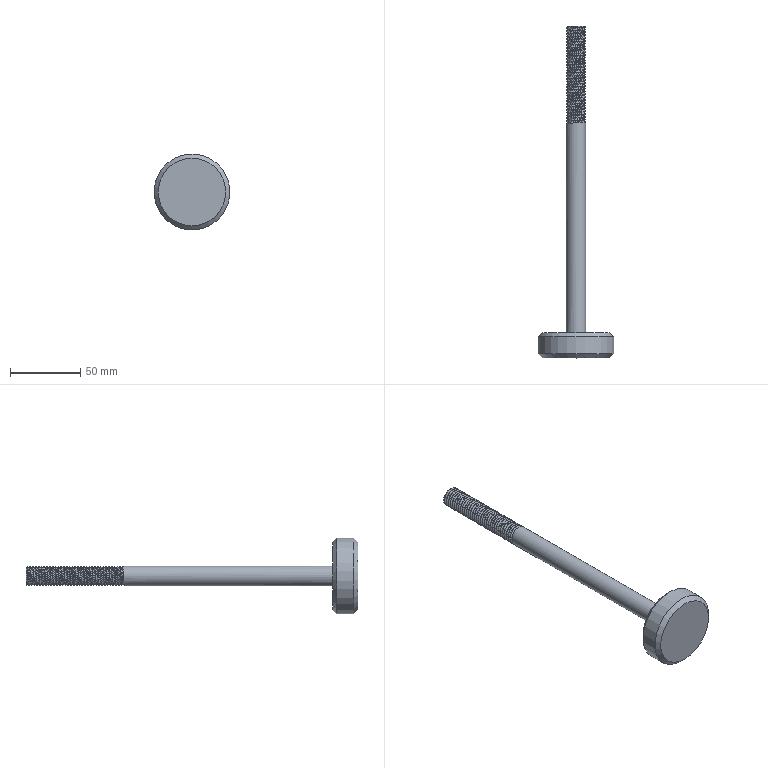Component | NX | SCREW_ROD | 1 solid | 46 faces | volume 71730 mm3 | cylinder 38 | plane 4 | cone 2 | spline 2 | commonest cylinder face diameters 14 x36 54 x1 12 x1